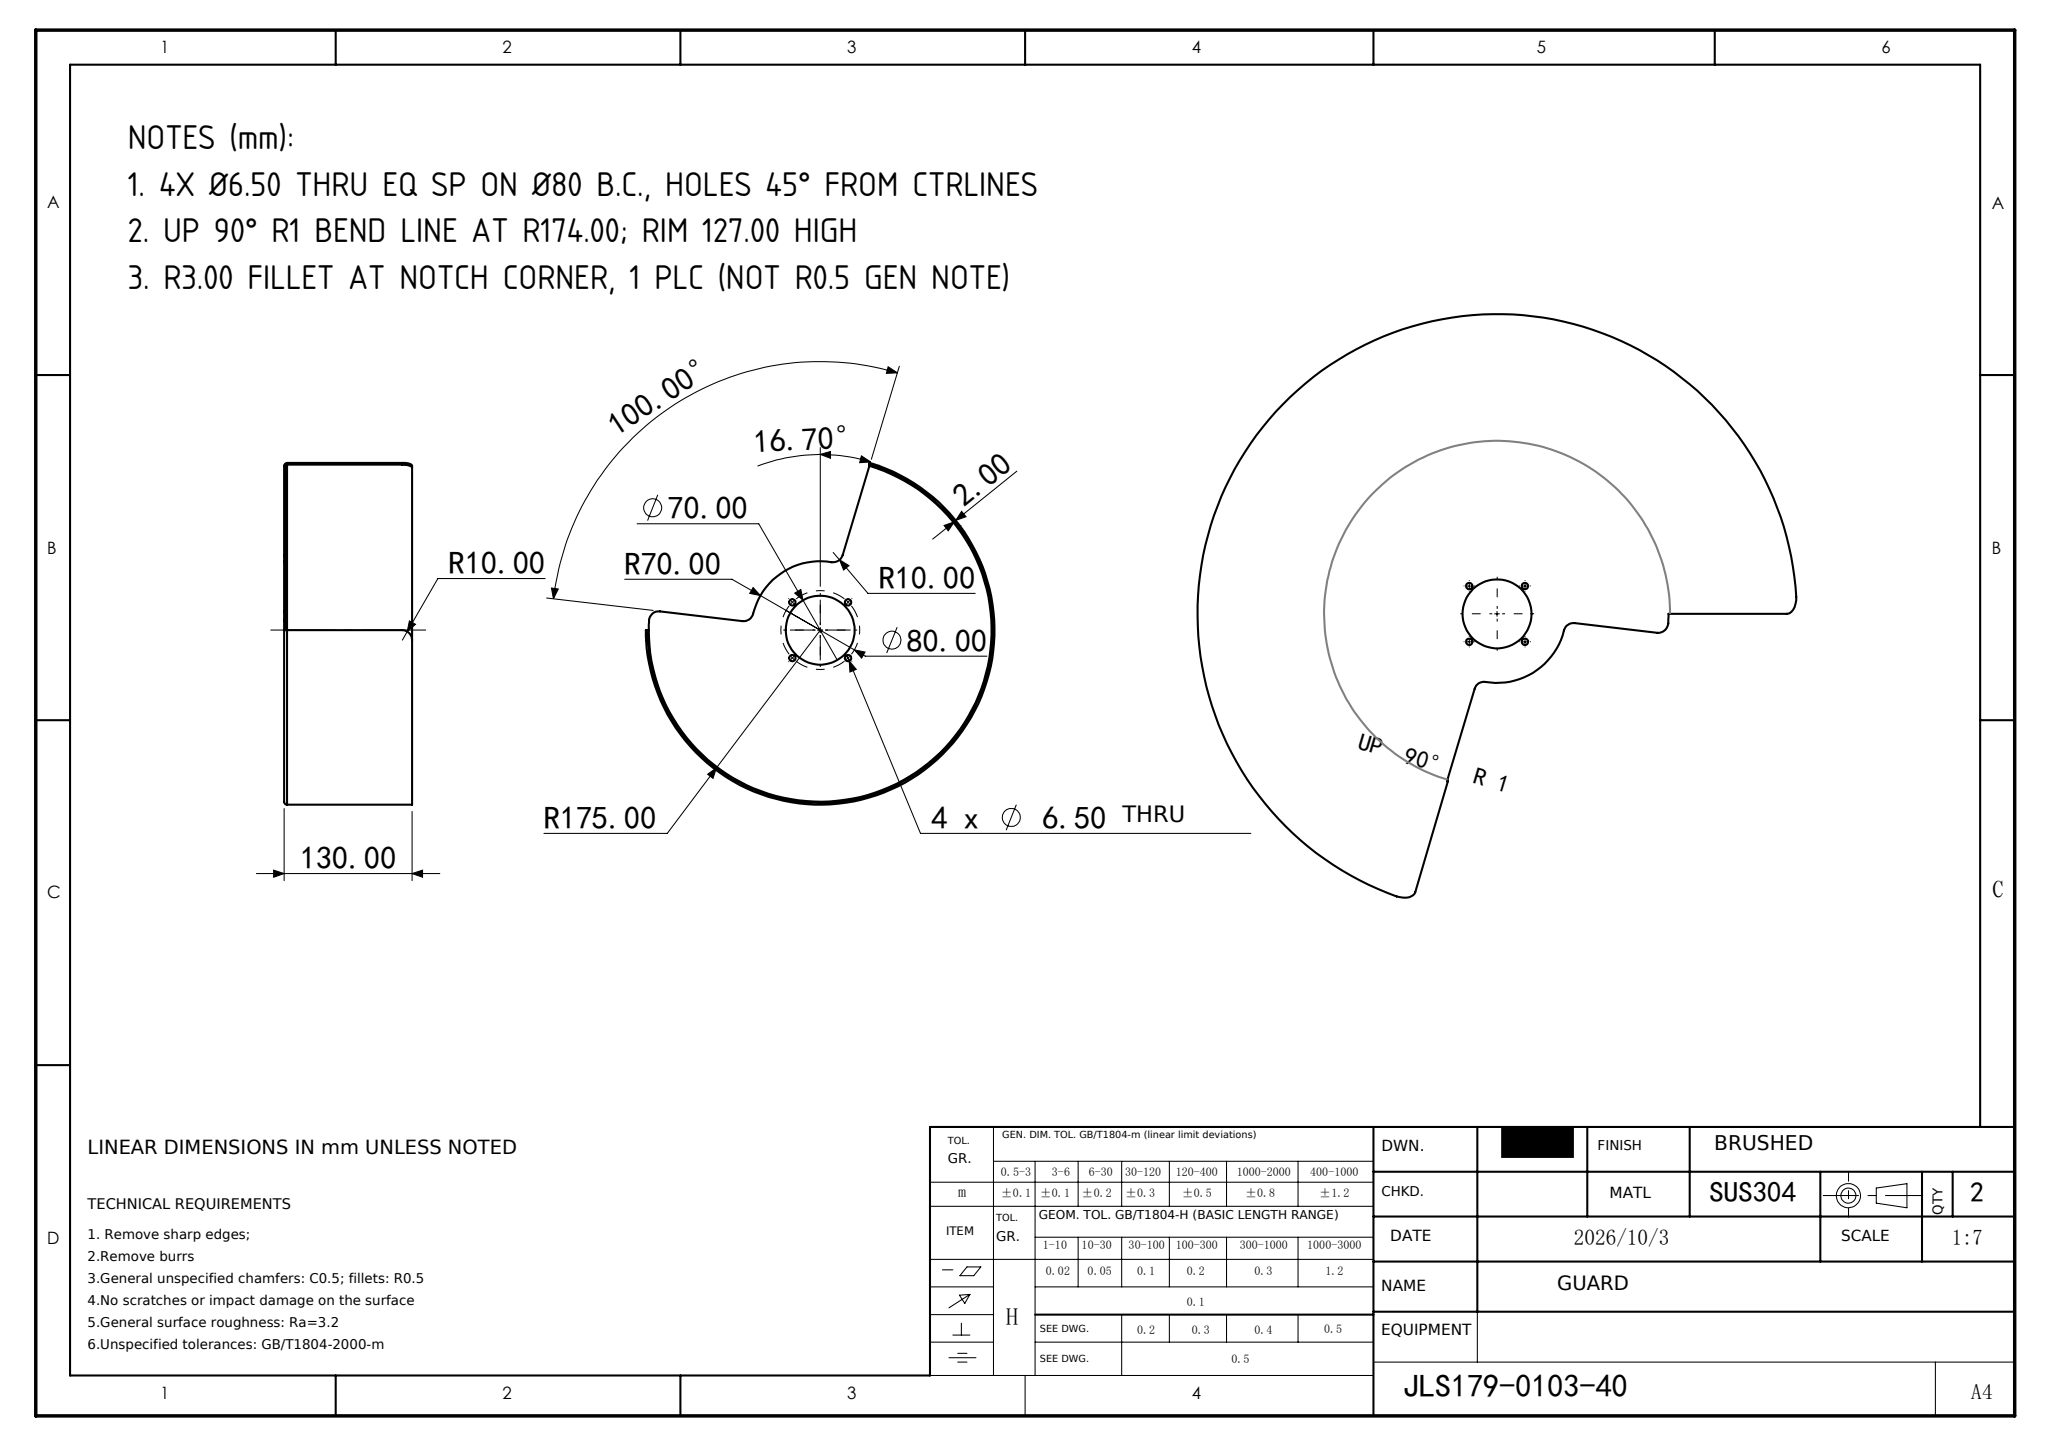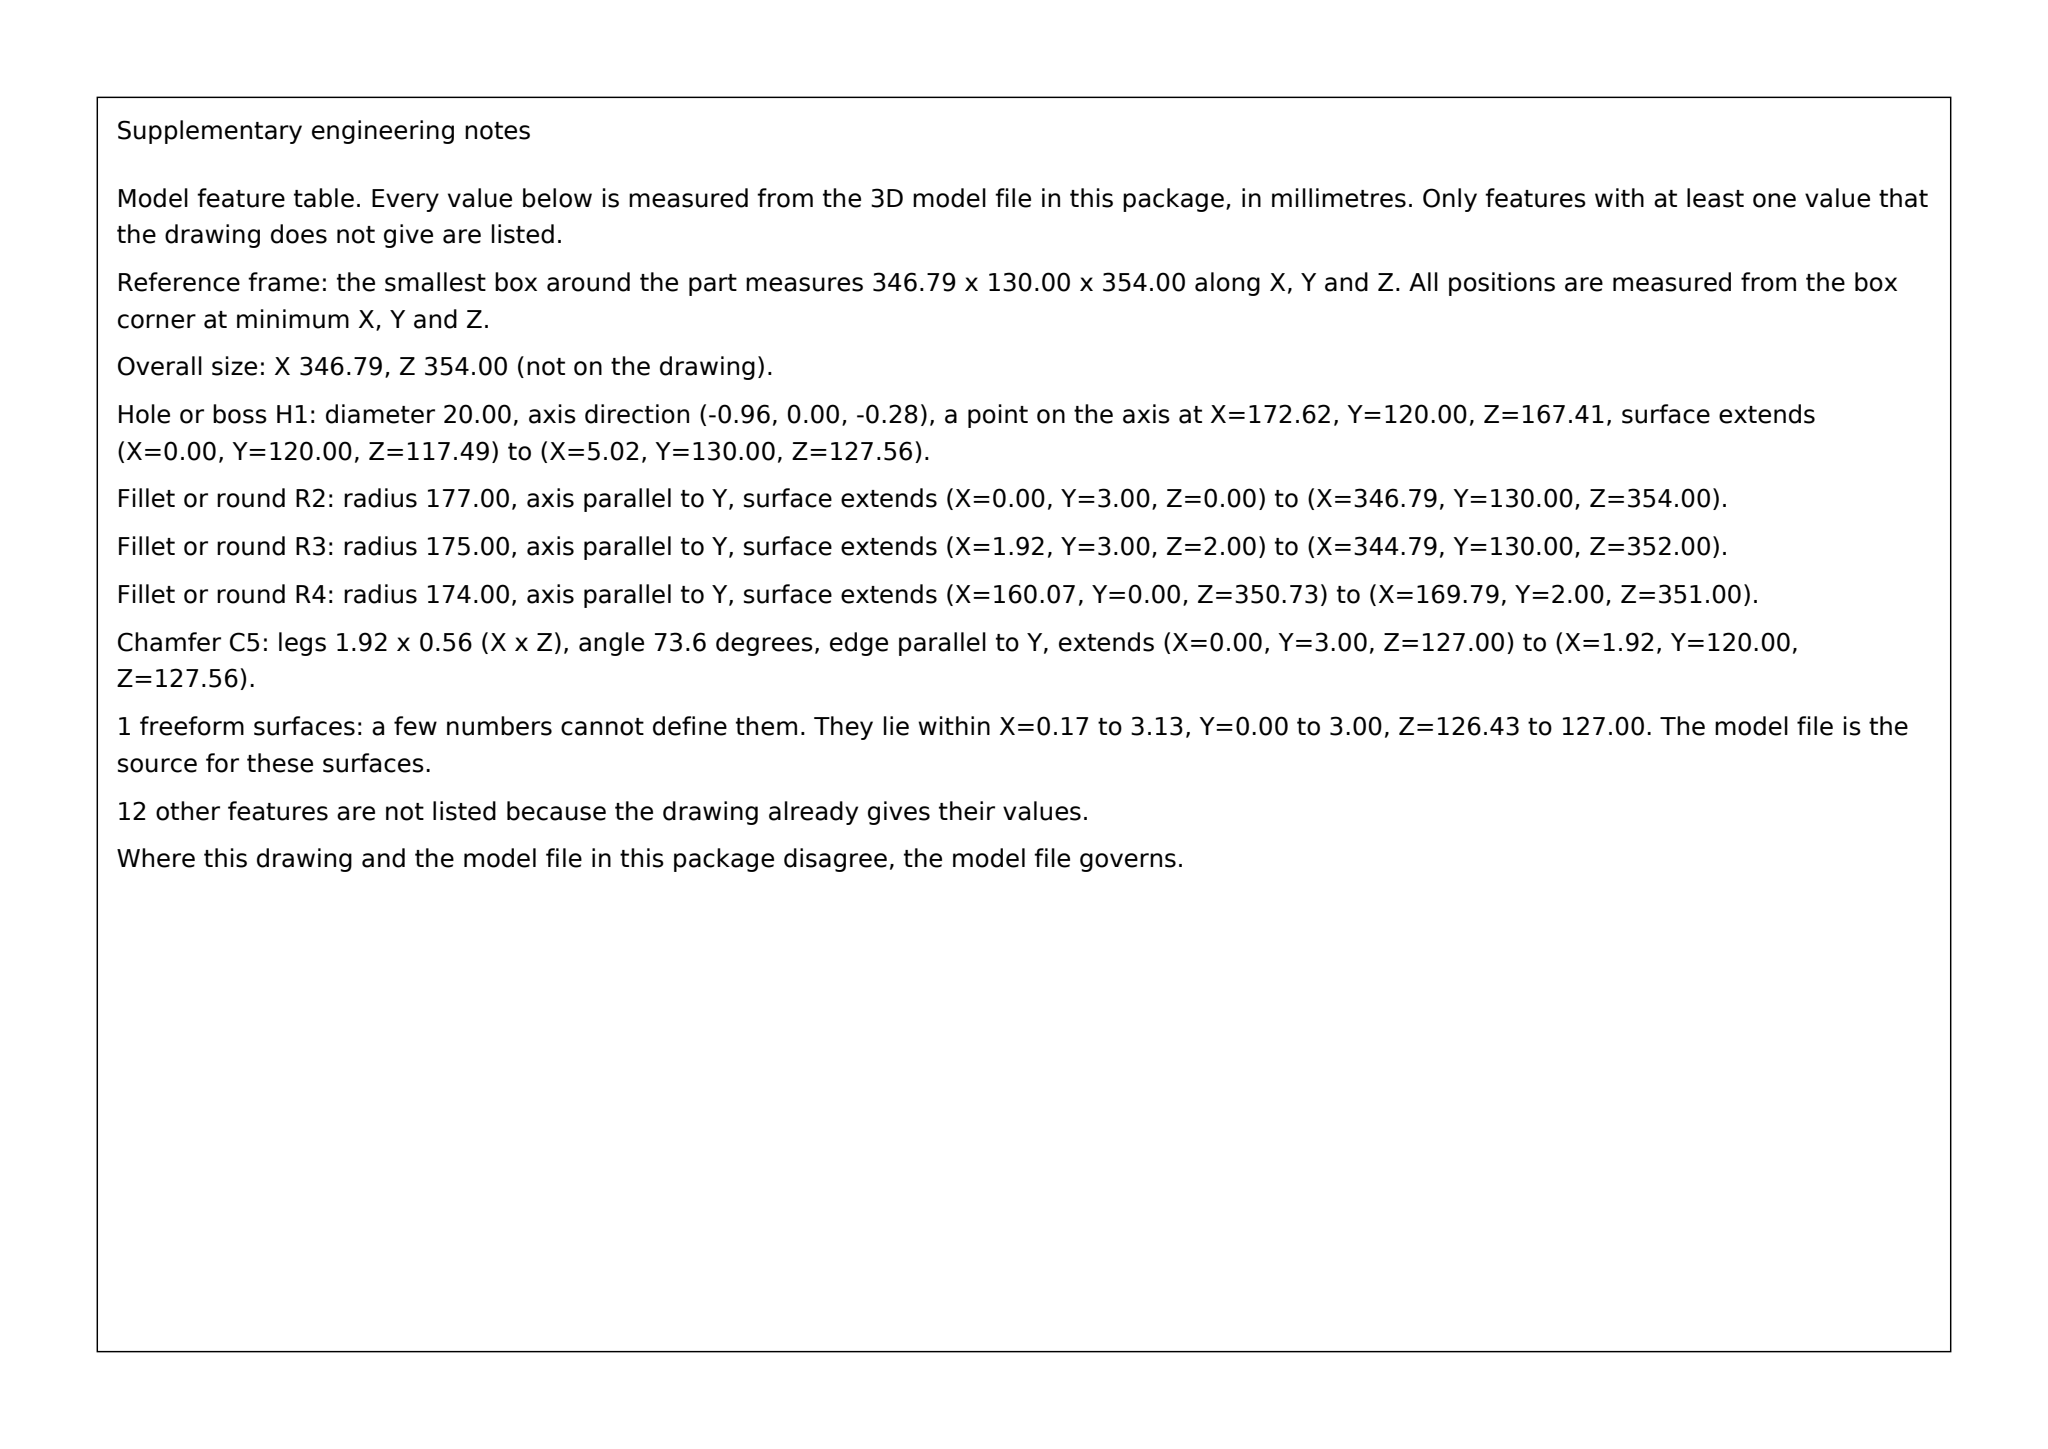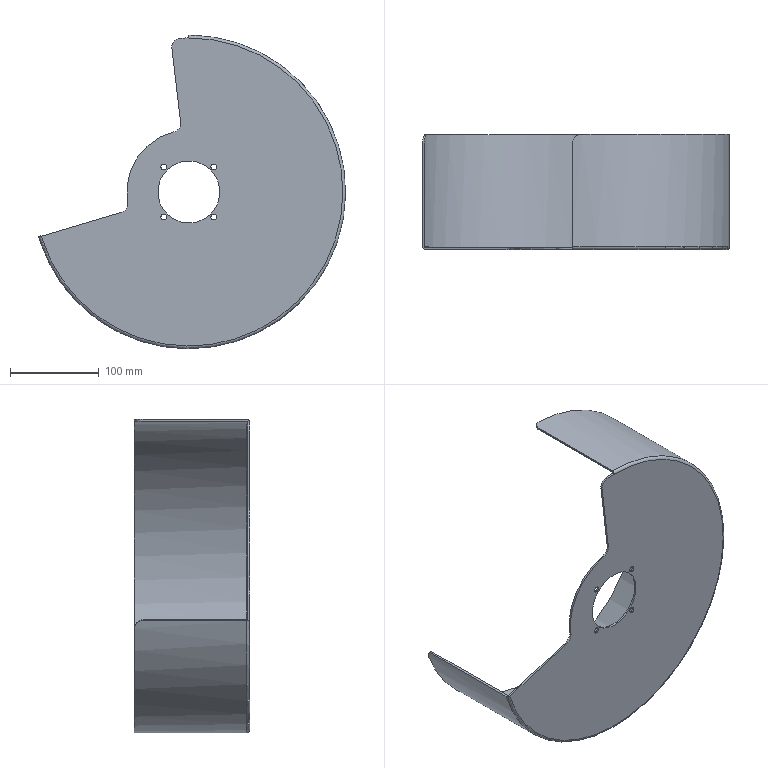Part | SolidWorks | mm | 1 solid | 31 faces | box 346.79 x 130 x 354 mm | volume 340648 mm3 | cylinder 19 | plane 9 | torus 2 | spline 1 | commonest cylinder face diameters 6.5 x8 20 x5 70 x2 350 x1 354 x1 348 x1 140 x1
Drawing notes:
4X Ø6.50 THRU EQ SP ON Ø80 B.C., HOLES 45° FROM CTRLINES | from the solid: 6.5 dia y-holes at x/z 155.31 & 211.88, 163.3 & 219.87 about ctr 183.6/191.58: ±28.285 each axis = Ø80 B.C., 90° apart, 45° off centerlines
UP 90° R1 BEND LINE AT R174.00; RIM 127.00 HIGH | from the solid: flat disc Ø348 (R174) at y 0.02-2.02; R1 fillet y 2.02-3.02 to rim ID Ø350; rim cyl Ø350/Ø354 length 127 (total 130.00)
R3.00 FILLET AT NOTCH CORNER, 1 PLC (NOT R0.5 GEN NOTE) | from the solid: fillet_radii [[1.0,1],[3.0,1]] - single R3.0 edge blend, only R1 called out on folded view